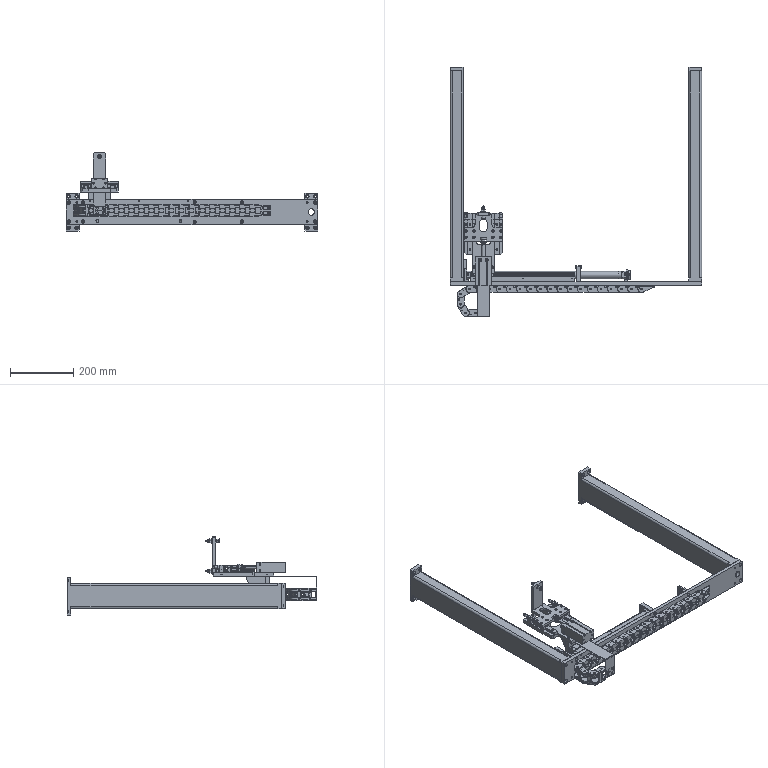Assembly | SolidWorks | mm | 74 component files | 74 solids | 4360 faces | box 795 x 790.5 x 247 mm | volume 3471055 mm3 | plane 2175 | cylinder 1835 | cone 314 | torus 28 | spline 8 | commonest cylinder face diameters 5.5 x192 22 x138 23 x130 3.4 x126 0.4 x126 2.444 x84 9.434 x84 5 x68
Bill of materials:
A0116 | 1 |  | Thick rectangular plate with an L-shaped side profile (a stepped ledge at one end), two chamfered corners on one long edge, one large and one medium through bore, a small face hole, and holes drilled into the narrow edge.
A0117 | 1 |  | Thin sheet-like L-shaped angle with a single rounded bend, a long flange and a shorter flange, and two small holes near the free end of the long flange.
A0131 | 1 |  | Plain rectangular block or thick bar with three round through holes on its main face in a triangular arrangement, one hole a different diameter from the other two.
A039 | 1 |  | Thick rectangular plate with two chamfered corners, a large through bore and a smaller bore, three small through holes along one edge, and three drilled holes in one narrow edge.
A066 | 1 |  | Long, thin flat bar with many through holes of several sizes spread along its length, including one larger hole near one end and small-hole groups near the ends and middle.
A067 | 2 |  | Long rectangular-section beam with a flat rectangular end plate at each end; the end plate has a large central bore, four corner through holes and two smaller blind holes; there are additional holes on the side near one end.
A091 | 1 |  | Long rectangular bar with a lengthwise rectangular groove along one face and a row of through holes of two or more sizes on the broad face.
1..2659899830.0 | 2 |  | Turned, stepped cylindrical part with a hexagonal collar near mid-length, a long cylindrical body, a slot across one end, and a small-diameter pin projecting from the other end with stepped shoulders.
A0106 | 2 |  | Solid rectangular block with one large round through hole near one end, passing through a pair of opposite faces.
A0110 | 1 |  | Rectangular plate with stepped faces (a transverse groove or step across one face and a small lip along the bottom edge), a pattern of about ten through holes including two larger bores, and two holes drilled into the top edge.
A0111 | 1 |  | Thick flat plate with a trapezoidal outline (one long diagonal edge, looking like a gusset), with two drilled holes in the top edge and two in the adjacent straight vertical edge.
A068 | 1 |  | Fork-shaped (U-slotted) thick plate: two parallel arms with a deep central slot that has rounded inner corners, a narrower tongue section at the base, chamfered shoulder corners, raised pads and steps at the arm ends, shallow lengthwise grooves along the arms, and many through holes of different sizes.
A069 | 1 |  | Flat plate with a roughly T-shaped outline. It has a central obround through-slot, eight round through-holes in two groups of four, and a T-shaped notch on one edge.
A070 | 1 |  | Axisymmetric spool or bushing shape: two flanges of different diameters joined by a smaller central hub, with a through-bore along the axis.
A071 | 1 |  | Thin rectangular plate with chamfered corners. It has two larger holes near the ends and two smaller holes near one end, beside notches in the long edges.
1.0.009603 | 1 |  | Rectangular block with two parallel narrow grooves running along its length. It has several holes on its faces and keyhole-like notches at the edges.
3..0..0.2 | 1 |  | Headed pin: a flat round disk head on a long cylindrical shank, which steps down to a smaller-diameter end section.
4..050.63 | 1 |  | Hexagonal prism with a large central round bore and chamfered (curved-edge) corners. Its shape matches a hex nut.
MANIFOLD_SOLID_BREP_100 | 2 |  | Rectangular block with an open channel through its underside, giving an inverted-U end profile. It has four holes on top and a seam line across the top near one end.
MANIFOLD_SOLID_BREP_99_1 | 2 |  | Straight bar of constant cross-section with three equally spaced holes through the top, rounded grooves along both sides, and chamfered corners.
1_2 | 2 |  | Elongated stepped turned part. It has a small flange at one end, cylindrical body sections, a knurled ring, and a hex section near the other end, with an axial bore at the flanged end.
2_2 | 2 |  | Axisymmetric stepped part: a cylindrical body with a rounded end and a small axial hole, a larger-diameter collar, a conical taper, a neck groove, and a small conical tip.
4_1 | 2 |  | Thin hexagonal ring with a large round bore and chamfered corners. Its shape matches a thin hex nut or lock-ring.
HGR15_1 | 1 |  | Long straight bar of constant cross-section with a shaped profile and a row of evenly spaced small holes along one side.
HGH15_2 | 1 |  | Rectangular prismatic block with a full-length open channel along one side, giving a C-shaped end profile. The top has a raised central section between lower stepped end sections. Generic shape resembles a linear-guide carriage block, but this is not confirmed.
10 | 1 |  | Link-like body made of two parallel stadium-shaped (obround) side plates joined by a central rectangular web, leaving an open rectangular window between the plates. At one end the plates are stepped outward (joggled). That end has a cylindrical boss or pin with a small bore; the other end has a plain through hole. Overall shape resembles a cable-carrier or chain link.
11 | 1 |  | Looks the same as the other link-like parts: two parallel stadium-shaped side plates joined by a central web with an open rectangular window, joggled plate ends, a cylindrical bored boss at one end and a through hole at the other.
12 | 1 |  | Looks the same as the other link-like parts: two parallel stadium-shaped side plates joined by a central web with an open rectangular window, joggled plate ends, a cylindrical bored boss at one end and a through hole at the other.
13 | 1 |  | Looks the same as the other link-like parts: two parallel stadium-shaped side plates joined by a central web with an open rectangular window, joggled plate ends, a cylindrical bored boss at one end and a through hole at the other.
14 | 1 |  | Looks the same as the other link-like parts: two parallel stadium-shaped side plates joined by a central web with an open rectangular window, joggled plate ends, a cylindrical bored boss at one end and a through hole at the other.
15 | 1 |  | Looks the same as the other link-like parts: two parallel stadium-shaped side plates joined by a central web with an open rectangular window, joggled plate ends, a cylindrical bored boss at one end and a through hole at the other.
16 | 1 |  | Looks the same as the other link-like parts: two parallel stadium-shaped side plates joined by a central web with an open rectangular window, joggled plate ends, a cylindrical bored boss at one end and a through hole at the other.
17 | 1 |  | Looks the same as the other link-like parts: two parallel stadium-shaped side plates joined by a central web with an open rectangular window, joggled plate ends, a cylindrical bored boss at one end and a through hole at the other.
18 | 1 |  | Looks the same as the other link-like parts: two parallel stadium-shaped side plates joined by a central web with an open rectangular window, joggled plate ends, a cylindrical bored boss at one end and a through hole at the other.
19 | 1 |  | Looks the same as the other link-like parts: two parallel stadium-shaped side plates joined by a central web with an open rectangular window, joggled plate ends, a cylindrical bored boss at one end and a through hole at the other.
20 | 1 |  | Looks the same as the other link-like parts: two parallel stadium-shaped side plates joined by a central web with an open rectangular window, joggled plate ends, a cylindrical bored boss at one end and a through hole at the other.
21 | 1 |  | Link-like frame: two parallel obround side plates joined by a central rectangular web, with a through-hole at one end and a short hollow cylindrical boss at the other.
22 | 1 |  | Link-like frame: two parallel obround side plates joined by a central rectangular web, with a through-hole at one end and a short hollow cylindrical boss at the other.
34 | 1 |  | Bent L-bracket: a tapered, teardrop-shaped flat flange with a round hole at its rounded end, and a perpendicular rectangular tab with two round holes rising from its straight edge.
35 | 1 |  | Bent L-bracket with a tapered teardrop flange and a perpendicular two-hole tab. Plan profile matches unnamed part, but the tab is bent the opposite way.
36 | 1 |  | Bent L-bracket: tapered teardrop flange with a central hole and several perimeter notches at the rounded end, plus a perpendicular two-hole tab along the flange's straight edge.
37 | 1 |  | Bent L-bracket with a notched teardrop flange and a perpendicular two-hole tab. Plan profile matches unnamed part, but the tab is bent the opposite way.
6 | 5 |  | Link-like frame: two parallel obround side plates joined by a central rectangular web, with a through-hole at one end and a short hollow cylindrical boss at the other.
7 | 1 |  | Link-like frame: two parallel obround side plates joined by a central rectangular web, with a through-hole at one end and a short hollow cylindrical boss at the other.
8 | 1 |  | Link-like frame: two parallel obround side plates joined by a central rectangular web, with a through-hole at one end and a short hollow cylindrical boss at the other.
9 | 1 |  | Link-like frame: two parallel obround side plates joined by a central rectangular web, with a through-hole at one end and a short hollow cylindrical boss at the other.
Mirror_A0116 | 1 |  | Thick rectangular plate with two chamfered corners on one long edge and three round through-holes of different sizes in the face. A stepped, L-shaped side profile forms a thicker lip along one end.
RMS20X400_0_Barrel | 1 |  | Straight thin-walled round tube with plain square-cut ends.
RMS20X50_Body | 1 |  | Rectangular prismatic block with a square end face containing a large circular bore along the long axis; concentric stepped rings or grooves surround the bore opening, and two small holes or features sit on the end face near the bore.
RMS20X50_FCV | 2 |  | Axially symmetric fitting-like body with a central hexagonal section and a cylindrical spigot on each side, chamfered at the outer ends, plus a central bore.
RMS20X50_Nut | 2 |  | Thin hexagonal nut-like ring with a large plain circular through-hole and chamfered corners on both faces.
RMS20X50_Piston | 1 |  | Solid stepped cylindrical shaft or pin: a large central cylinder with a smaller-diameter journal or stub at each end, a small shoulder step between them, and rounded or chamfered ends.
1 | 4 |  | Bolt-like part with a hexagonal head, a short cylindrical boss on the outer side of the head, a plain cylindrical shank with a chamfered tip, and a hexagonal socket recess in the shank end.
2 | 4 |  | Hexagonal nut-like body, thicker than part-02d4..., with a plain circular through-hole and chamfers on both faces.
Mates:
1. coincident | A066-2 face at (318.881, 0, 60) dir (0, 1, 0) | A067-6 face at (696.381, 0, 60) dir (0, -1, 0)
2. coincident | A066-2 face at (716.381, -12, 100) dir (1, 0, 0) | A067-6 face at (716.381, 12, 26) dir (1, 0, 0)
3. coincident | A066-2 face at (716.381, -12, 20) dir (0, 0, -1) | A067-6 face at (682.381, 12, 20) dir (0, 0, -1)
4. coincident | A066-2 face at (318.881, 0, 60) dir (0, 1, 0) | A067-7 face at (-58.619, 0, 60) dir (0, -1, 0)
5. coincident | A066-2 face at (716.381, -12, 100) dir (0, 0, 1) | A067-7 face at (-72.619, 12, 100) dir (0, 0, 1)
6. coincident | A066-2 face at (-78.619, -12, 100) dir (-1, 0, 0) | A067-7 face at (-78.619, 12, 26) dir (-1, 0, 0)
7. coincident | HandlingMechanism-2/A0110-1 face at (25.881, 41, 71.5) dir (0, -1, 0) | RMS_20X400_03-1/RMS20X50_Body-1 face at (60.881, 41, 22) dir (0, 1, 0)
8. coincident | HandlingMechanism-2/A0110-1 face at (60.881, 51.5, 20) dir (1, 0, 0) | RMS_20X400_03-1/RMS20X50_Body-1 face at (60.881, 40.5, 61) dir (1, 0, 0)
9. concentric | RMS_20X400_03-1/RMS20X400_0_Barrel-1 face at (463.381, 21, 41.5) dir (-1, 0, 0) r 11.5 | A0116-1 face at (-32.619, 21, 41.5) dir (1, 0, 0) r 10
10. coincident | A066-2 face at (318.881, 0, 60) dir (0, 1, 0) | A0116-1 face at (-20.619, 0, 100) dir (0, -1, 0)
11. coincident | RMS_20X400_03-1/RMS20X50_FCV-1 face at (-27.619, 21, 31.5) dir (-1, 0, 0) | A0116-1 face at (-27.619, 38.5, 100) dir (1, 0, 0)
12. concentric | RMS_20X400_03-1/RMS20X400_0_Barrel-1 face at (463.381, 21, 41.5) dir (-1, 0, 0) r 11.5 | Mirror_A0116-3 face at (483.381, 21, 41.5) dir (-1, 0, 0) r 10
13. coincident | A0116-1 face at (-32.619, 0, 20) dir (0, 0, -1) | Mirror_A0116-3 face at (483.381, 0, 20) dir (0, 0, -1)
14. coincident | RMS_20X400_03-1/RMS20X50_FCV-2 face at (478.381, 21, 51.5) dir (1, 0, 0) | Mirror_A0116-3 face at (478.381, 38.5, 100) dir (-1, 0, 0)
15. distance | HandlingMechanism-2/A071-1 plane at (25.881, 208.5, 187) dir (-1, 0, 0) | A067-7 face at (-38.619, 12, 26) dir (1, 0, 0)
16. distance | HandlingMechanism-2/A0110-1 face at (60.881, 51.5, 20) dir (0, 0, -1) | RMS_20X400_03-1/RMS20X50_Body-1 face at (60.881, 1.5, 21.5) dir (0, 0, -1)
17. distance | A066-2 face at (716.381, -12, 20) dir (0, 0, -1) | RMS_20X400_03-1/RMS20X50_Body-1 face at (60.881, 1.5, 21.5) dir (0, 0, -1)
18. coincident | A066-2 face at (318.881, -12, 60) dir (0, -1, 0) | MHPUS204-38-33-A-1/35-1 face at (568.833, -12, 81.7) dir (0, 1, 0)
19. distance | MHPUS204-38-33-A-1 plane at (-41.387, -64.533, 65) dir (0, 0, 1) | HandlingMechanism-2/CDU25-40A-A93(0_0)-2/1.0.009603-1 face at (36.881, 78.5, 135) dir (0, 0, -1)
20. coincident | HandlingMechanism-2/A068-1 face at (25.881, 120.5, 123) dir (0, 0, -1) | A0117-1 face at (45.881, -111.5, 123) dir (0, 0, 1)
21. coincident | HandlingMechanism-2/A0110-1 face at (25.881, 39.5, 71.5) dir (0, -1, 0) | A0117-1 face at (45.881, 39.5, 123) dir (0, 1, 0)
22. width | A0117-1 face at (45.881, -110, 121) dir (1, 0, 0) | A0117-1 face at (5.881, -109.5, 121) dir (-1, 0, 0) | HandlingMechanism-2/A068-1 face at (60.881, 24.5, 115) dir (1, 0, 0) | HandlingMechanism-2/A068-1 face at (-9.119, 24.5, 115) dir (-1, 0, 0)
23. concentric | Mirror_A0116-3 face at (483.381, 23.5, 75) dir (1, 0, 0) r 2.5 | USTH5-15-1/1-1 face at (484.735, 23.5, 75) dir (1, 0, 0) r 2.5
24. coincident | Mirror_A0116-3 face at (483.381, 0, 100) dir (1, 0, 0) | USTH5-15-1/2-1 face at (483.381, 21.5, 75) dir (-1, 0, 0)
25. concentric | A0116-1 face at (-32.619, 23.5, 75) dir (-1, 0, 0) r 2.5 | USTH5-15-2/1-1 face at (-33.974, 23.5, 75) dir (-1, 0, 0) r 2.5
26. coincident | A0116-1 face at (-32.619, 0, 100) dir (-1, 0, 0) | USTH5-15-2/2-1 face at (-32.619, 22.736, 76.848) dir (1, 0, 0)
27. coincident | A066-2 face at (318.881, 0, 60) dir (0, 1, 0) | A039-1 face at (333.381, 0, 100) dir (0, -1, 0)
28. distance | A039-1 face at (333.381, 25.5, 60) dir (1, 0, 0) | Mirror_A0116-3 face at (478.381, 38.5, 100) dir (-1, 0, 0)
29. coincident | A066-2 face at (716.381, -12, 100) dir (0, 0, 1) | A039-1 face at (333.381, 51, 100) dir (0, 0, 1)
30. coincident | USTH5-15-3/1-1 face at (316.381, 47.5, 90) dir (-1, 0, 0) | USTH5-15-4/1-1 face at (316.381, 47.5, 30) dir (-1, 0, 0)
31. concentric | A039-1 face at (333.381, 46, 30) dir (1, 0, 0) r 2.5 | USTH5-15-4/1-1 face at (328.635, 46, 30) dir (1, 0, 0) r 2.5
32. concentric | A039-1 face at (333.381, 46, 90) dir (1, 0, 0) r 2.5 | USTH5-15-3/1-1 face at (328.635, 46, 90) dir (1, 0, 0) r 2.5
33. coincident | A039-1 face at (321.381, 25.5, 60) dir (-1, 0, 0) | USTH5-15-3/1-1 face at (321.381, 49.65, 90) dir (1, 0, 0)
34. coincident | HandlingMechanism-2/A0110-1 face at (25.881, 41, 71.5) dir (0, -1, 0) | HGH15CA-1/HGH15_2-1 face at (6.181, 41, 92) dir (0, 1, 0)
35. coincident | HandlingMechanism-2/A0110-1 face at (60.881, 41, 66) dir (0, 0, 1) | HGH15CA-1/HGH15_2-1 face at (6.181, 35, 66) dir (0, 0, -1)
36. width | HGH15CA-1/HGH_15_ASM_3_ASM-1/HGR15_1-1 face at (315.381, 21.635, 76.177) dir (1, 0, 0) | HGH15CA-1/HGH_15_ASM_3_ASM-1/HGR15_1-1 face at (-14.619, 28, 83) dir (-1, 0, 0) | A0116-1 face at (-20.619, 8, 100) dir (1, 0, 0) | A039-1 face at (321.381, 25.5, 60) dir (-1, 0, 0)
37. width | HGH15CA-1/HGH15_2-1 face at (56.581, 28, 83) dir (1, 0, 0) | HGH15CA-1/HGH15_2-1 face at (-4.819, 28, 83) dir (-1, 0, 0) | HandlingMechanism-2/A0110-1 face at (-9.119, 51.5, 20) dir (-1, 0, 0) | HandlingMechanism-2/A0110-1 face at (60.881, 51.5, 20) dir (1, 0, 0)
38. coincident | A066-2 face at (318.881, 0, 60) dir (0, 1, 0) | A091-2 face at (150.381, 0, 83) dir (0, -1, 0)
39. coincident | HGH15CA-1/HGH_15_ASM_3_ASM-1/HGR15_1-1 face at (-14.619, 13.7, 75.5) dir (0, 0, -1) | A091-2 face at (-14.619, 13, 75.5) dir (0, 0, 1)
40. coincident | HGH15CA-1/HGH_15_ASM_3_ASM-1/HGR15_1-1 face at (315.381, 21.635, 76.177) dir (1, 0, 0) | A091-2 face at (315.381, 15, 100) dir (1, 0, 0)
41. coincident | A067-7 face at (-38.619, 12, 26) dir (1, 0, 0) | A0131-1 face at (-38.619, 56, 60) dir (-1, 0, 0)
42. coincident | A067-7 face at (-72.619, 12, 20) dir (0, 0, -1) | A0131-1 face at (-28.619, 41, 20) dir (0, 0, -1)
43. coincident | HandlingMechanism-2/A0110-1 face at (25.881, 41, 71.5) dir (0, -1, 0) | A0131-1 face at (-28.619, 41, 20) dir (0, -1, 0)
44. coincident | A039-1 face at (333.381, 25.5, 60) dir (1, 0, 0) | USTH5-15-3/2-1 face at (333.381, 44, 90) dir (-1, 0, 0)
45. concentric | A039-1 face at (333.381, 46, 90) dir (1, 0, 0) r 2.5 | USTH5-15-3/2-1 face at (336.581, 46, 90) dir (-1, 0, 0) r 2.5
46. coincident | A039-1 face at (333.381, 25.5, 60) dir (1, 0, 0) | USTH5-15-4/2-1 face at (333.381, 44, 30) dir (-1, 0, 0)
47. concentric | A039-1 face at (333.381, 46, 30) dir (1, 0, 0) r 2.5 | USTH5-15-4/2-1 face at (336.581, 46, 30) dir (-1, 0, 0) r 2.5
48. parallel | A069-1 face at (-48.143, -85.976, 28) dir (0, -1, 0) | A071-1 face at (11.857, -82.976, 58) dir (0, 1, 0)
49. width | A071-1 face at (-8.143, -92.976, 118) dir (-1, 0, 0) | A071-1 face at (31.857, -92.976, 118) dir (1, 0, 0) | A068-1 face at (-10.643, -90.976, -6) dir (1, 0, 0) | A068-1 face at (34.357, -90.976, -6) dir (-1, 0, 0)
50. coincident | A071-1 face at (11.857, -92.976, 58) dir (0, -1, 0) | MVPTN2-1/4_1-1 face at (9.652, -92.976, 12.718) dir (0, 1, 0)
51. concentric | A071-1 face at (11.857, -92.976, 10) dir (0, -1, 0) r 6 | MVPTN2-1/1_2-1 face at (11.857, -89.976, 10) dir (0, -1, 0) r 6
52. concentric | A071-1 face at (11.857, -92.976, 106) dir (0, -1, 0) r 6 | MVPTN2-3/1_2-1 face at (11.857, -89.976, 106) dir (0, -1, 0) r 6
53. coincident | A068-1 face at (11.857, 5.024, 4) dir (0, 0, 1) | A0106-1 face at (-43.143, -64.976, 4) dir (0, 0, -1)
54. coincident | A068-1 face at (-48.143, 101.024, 6) dir (-1, 0, 0) | A0106-1 face at (-48.143, -58.976, 4) dir (-1, 0, 0)
55. coincident | A068-1 face at (11.857, 5.024, 4) dir (0, 0, 1) | A0106-2 face at (66.857, -64.976, 4) dir (0, 0, -1)
56. coincident | A068-1 face at (71.857, 101.024, 6) dir (1, 0, 0) | A0106-2 face at (71.857, -58.976, 4) dir (1, 0, 0)
57. coincident | A068-1 face at (-48.143, -58.976, 4) dir (0, -1, 0) | A0106-2 face at (61.857, -58.976, 4) dir (0, 1, 0)
58. coincident | A068-1 face at (-48.143, -58.976, 4) dir (0, -1, 0) | A0106-1 face at (-48.143, -58.976, 4) dir (0, 1, 0)
59. coincident | A069-1 face at (1.857, -13.976, 13) dir (0, 1, 0) | A070-1 face at (11.857, -13.976, 22) dir (0, -1, 0)
60. concentric | A0106-2 face at (66.857, -58.976, 23) dir (0, 1, 0) r 4 | 1..2659899830.0-1 face at (66.857, -70.076, 23) dir (0, -1, 0) r 4
61. coincident | A0106-2 face at (61.857, -70.976, 4) dir (0, -1, 0) | 1..2659899830.0-1 face at (66.857, -70.976, 23) dir (0, 1, 0)
62. concentric | A0106-1 face at (-43.143, -58.976, 23) dir (0, 1, 0) r 4 | RB0805(0)-1/1..2659899830.0-1 face at (-43.143, -70.076, 23) dir (0, -1, 0) r 4
63. coincident | A0106-1 face at (-48.143, -70.976, 4) dir (0, -1, 0) | RB0805(0)-1/1..2659899830.0-1 face at (-43.143, -70.976, 23) dir (0, 1, 0)
64. distance | A071-1 face at (31.857, -92.976, 118) dir (0, 0, 1) | A069-1 face at (11.857, -44.476, 28) dir (0, 0, 1)
65. coincident | A068-1 face at (11.857, 5.024, -6) dir (0, 0, -1) | A0110-1 face at (-23.143, 74.024, -6) dir (0, 0, 1)
66. width | A069-1 face at (-48.143, -2.976, 28) dir (-1, 0, 0) | A069-1 face at (71.857, -2.976, 28) dir (1, 0, 0) | A068-1 face at (71.857, 101.024, 6) dir (1, 0, 0) | A068-1 face at (-48.143, 101.024, 6) dir (-1, 0, 0)
67. concentric | A070-1 face at (11.857, 1.024, 22) dir (0, -1, 0) r 9.75 | CDU25-40A-A93(0_0)-2/3..0..0.2-1 face at (11.857, -2.592, 22) dir (0, 1, 0) r 4
68. coincident | A070-1 face at (11.857, 1.024, 22) dir (0, 1, 0) | CDU25-40A-A93(0_0)-2/4..050.63-1 face at (10.204, 1.024, 17.017) dir (0, -1, 0)
69. coincident | MGN15C-5/MANIFOLD_SOLID_BREP_100-2 face at (-46.643, -37.826, 19.75) dir (0, 0, 1) | MGN15C-6/MANIFOLD_SOLID_BREP_100-2 face at (38.357, -37.826, 19.75) dir (0, 0, 1)
70. coincident | A068-1 face at (11.857, 5.024, 4) dir (0, 0, 1) | MGN15C-5/MANIFOLD_SOLID_BREP_99_1-1 face at (-38.143, -70.976, 4) dir (0, 0, -1)
71. coincident | A068-1 face at (-38.143, 39.024, 4) dir (1, 0, 0) | MGN15C-5/MANIFOLD_SOLID_BREP_99_1-1 face at (-38.143, -70.976, 9) dir (-1, 0, 0)
72. coincident | A068-1 face at (61.857, 39.024, 4) dir (-1, 0, 0) | MGN15C-6/MANIFOLD_SOLID_BREP_99_1-1 face at (61.857, -70.976, 4) dir (1, 0, 0)
73. coincident | A069-1 face at (11.857, -44.476, 20) dir (0, 0, -1) | MGN15C-5/MANIFOLD_SOLID_BREP_100-2 face at (-46.643, -45.526, 20) dir (0, 0, 1)
74. coincident | MGN15C-5/MANIFOLD_SOLID_BREP_100-2 face at (-14.643, -3.426, 12) dir (0, 1, 0) | MGN15C-6/MANIFOLD_SOLID_BREP_100-2 face at (70.357, -3.426, 12) dir (0, 1, 0)
75. coincident | A071-1 face at (11.857, -92.976, 58) dir (0, -1, 0) | MVPTN2-3/4_1-1 face at (11.669, -92.976, 102.505) dir (0, 1, 0)
76. width | A0110-1 face at (-23.143, 74.024, -109) dir (-1, 0, 0) | A0110-1 face at (46.857, 74.024, -109) dir (1, 0, 0) | A068-1 face at (46.857, 101.024, -14) dir (1, 0, 0) | A068-1 face at (-23.143, 101.024, -14) dir (-1, 0, 0)
77. width | A0111-2 face at (5.857, 44.024, -48.5) dir (-1, 0, 0) | A0111-2 face at (17.857, 44.024, -48.5) dir (1, 0, 0) | A0110-1 face at (-23.143, 74.024, -109) dir (-1, 0, 0) | A0110-1 face at (46.857, 74.024, -109) dir (1, 0, 0)
78. distance | CDU25-40A-A93(0_0)-2/1.0.009603-1 face at (11.857, 47.024, 22) dir (0, -1, 0) | A068-1 face at (-48.143, -90.976, 6) dir (0, -1, 0)
79. coincident | A068-1 face at (11.857, 5.024, 6) dir (0, 0, 1) | CDU25-40A-A93(0_0)-2/1.0.009603-1 face at (25.857, 47.024, 6) dir (0, 0, -1)
80. width | CDU25-40A-A93(0_0)-2/1.0.009603-1 face at (-13.143, 47.024, 38) dir (-1, 0, 0) | CDU25-40A-A93(0_0)-2/1.0.009603-1 face at (36.857, 47.024, 6) dir (1, 0, 0) | A068-1 face at (71.857, 101.024, 6) dir (1, 0, 0) | A068-1 face at (-48.143, 101.024, 6) dir (-1, 0, 0)
81. coincident | A069-1 face at (30.857, -82.976, 38) dir (0, -1, 0) | A071-1 face at (11.857, -82.976, 58) dir (0, 1, 0)
82. coincident | A0110-1 face at (11.857, 74.024, -57.5) dir (0, -1, 0) | A0111-2 face at (17.857, 74.024, -91) dir (0, 1, 0)
83. coincident | A068-1 face at (11.857, 5.024, -6) dir (0, 0, -1) | A0111-2 face at (17.857, 14.024, -6) dir (0, 0, 1)
84. width | A0111-2 face at (17.857, 44.024, -48.5) dir (1, 0, 0) | A0111-2 face at (5.857, 44.024, -48.5) dir (-1, 0, 0) | A0110-1 face at (-23.143, 74.024, -109) dir (-1, 0, 0) | A0110-1 face at (46.857, 74.024, -109) dir (1, 0, 0)
85. distance | A0110-1 face at (11.857, 86.024, -57.5) dir (0, 1, 0) | A068-1 face at (71.857, 39.024, -14) dir (0, 1, 0)
86. concentric | A069-1 face at (66.857, -34.476, 28) dir (0, 0, 1) r 2.15 | MGN15C-6/MANIFOLD_SOLID_BREP_100-2 face at (66.857, -34.476, 20) dir (0, 0, -1) r 1.5
87. concentric | A069-1 face at (66.857, -14.476, 28) dir (0, 0, 1) r 2.15 | MGN15C-6/MANIFOLD_SOLID_BREP_100-2 face at (66.857, -14.476, 20) dir (0, 0, -1) r 1.5
88. concentric | A069-1 face at (-43.143, -34.476, 28) dir (0, 0, 1) r 2.15 | MGN15C-5/MANIFOLD_SOLID_BREP_100-2 face at (-43.143, -34.476, 20) dir (0, 0, -1) r 1.5
89. concentric | A069-1 face at (-43.143, -14.476, 28) dir (0, 0, 1) r 2.15 | MGN15C-5/MANIFOLD_SOLID_BREP_100-2 face at (-43.143, -14.476, 20) dir (0, 0, -1) r 1.5
90. coincident | A068-1 face at (-48.143, 39.024, -14) dir (0, 1, 0) | MGN15C-5/MANIFOLD_SOLID_BREP_99_1-1 face at (-29.643, 39.024, 4) dir (0, 1, 0)
91. coincident | A068-1 face at (71.857, 39.024, -14) dir (0, 1, 0) | MGN15C-6/MANIFOLD_SOLID_BREP_99_1-1 face at (55.357, 39.024, 4) dir (0, 1, 0)
92. concentric | 3..0..0.2-1 face at (-38.432, 42.862, 93.705) dir (0, 0, -1) r 4 | 4..050.63-1 face at (-38.432, 42.862, 87.588) dir (0, 0, -1) r 3.324
93. coincident | 3..0..0.2-1 edge at (-38.432, 42.862, 85.088) dir (0, 0, -1) r 4 | 4..050.63-1 face at (-38.432, 48.112, 85.088) dir (0, 0, -1)
94. concentric | 1.0.009603-1 face at (-38.432, 42.862, 27.213) dir (0, 0, -1) r 5 | 3..0..0.2-1 face at (-38.432, 42.862, 49.213) dir (0, 0, -1) r 5
95. distance | 3..0..0.2-1 face at (-30.196, 45.819, 14.338) dir (0, 0, 1) | 1.0.009603-1 face at (-38.432, 49.112, -30.662) dir (0, 0, 1)
96. coincident | MANIFOLD_SOLID_BREP_99_1-1 face at (21.631, 13, 143.222) dir (0, 1, 0) | MANIFOLD_SOLID_BREP_100-2 face at (21.631, 13, 160.355) dir (0, -1, 0)
97. width | MANIFOLD_SOLID_BREP_100-2 face at (-1.869, 7, 126.405) dir (-1, 0, 0) | MANIFOLD_SOLID_BREP_100-2 face at (30.131, 19, 126.405) dir (1, 0, 0) | MANIFOLD_SOLID_BREP_99_1-1 face at (21.631, 3, 143.222) dir (1, 0, 0) | MANIFOLD_SOLID_BREP_99_1-1 face at (6.631, 8, 143.222) dir (-1, 0, 0)
98. concentric | 1_2-1 face at (8.638, 25.061, 13.204) dir (0, -1, 0) r 6 | 4_1-1 face at (8.638, 20.061, 13.204) dir (0, 1, 0) r 5.458
99. coincident | 1_2-1 face at (11.638, 18.061, 13.204) dir (0, 1, 0) | 4_1-1 face at (12.138, 18.061, 13.204) dir (0, -1, 0)
100. concentric | 1_2-1 face at (8.638, 6.561, 13.204) dir (0, -1, 0) r 2 | 2_2-1 face at (8.638, 6.411, 13.204) dir (0, -1, 0) r 1.6
101. coincident | 1_2-1 face at (10.638, 4.561, 13.204) dir (0, -1, 0) | 2_2-1 face at (10.438, 4.561, 13.204) dir (0, 1, 0)
102. width | HGH15_2-1 face at (13.858, 7, 25.799) dir (1, 0, 0) | HGH15_2-1 face at (-20.142, 12, 25.799) dir (-1, 0, 0) | HGH_15_ASM_3_ASM-1/HGR15_1-1 face at (-10.642, -11.757, -79.451) dir (-1, 0, 0) | HGH_15_ASM_3_ASM-1/HGR15_1-1 face at (4.358, -14.3, -79.451) dir (1, 0, 0)
103. coincident | HGH_15_ASM_3_ASM-1/HGR15_1-1 face at (1.907, 0, -79.451) dir (0, 1, 0) | HGH15_2-1 face at (-8.191, 0, 25.799) dir (0, -1, 0)
104. coincident | 34-1 face at (567.22, 52.533, -16.7) dir (0, 1, 0) | 35-1 face at (610.22, 52.533, 16.7) dir (0, 1, 0)
105. concentric | 22-1 face at (567.22, 41.533, -14.7) dir (0, 0, 1) r 2.75 | 34-1 face at (567.22, 41.533, -16.7) dir (0, 0, -1) r 2.75
106. concentric | 22-1 face at (567.22, 41.533, 14.7) dir (0, 0, -1) r 2.75 | 35-1 face at (567.22, 41.533, 16.7) dir (0, 0, 1) r 2.75
107. concentric | 6-2 face at (-5.032, -6.773, 14.4) dir (0, 0, -1) r 2.75 | 6-3 face at (-5.032, -6.773, -20) dir (0, 0, -1) r 2.75
108. concentric | 6-2 face at (11, -34.467, -20.3) dir (0, 0, -1) r 2.75 | 6-4 face at (11, -34.467, 14.7) dir (0, 0, -1) r 2.75
109. concentric | 36-1 face at (43, -34.467, -15) dir (0, 0, -1) r 2.75 | 6-4 face at (43, -34.467, -20) dir (0, 0, -1) r 2.75
110. coincident | 6-2 face at (16.511, -43.987, 14.7) dir (0, 0, -1) | 6-4 face at (54, -34.467, 14.7) dir (0, 0, 1)
111. concentric | 6-1 face at (23.22, 41.533, -20) dir (0, 0, -1) r 2.75 | 6-5 face at (23.22, 41.533, -14.7) dir (0, 0, 1) r 2.75
112. coincident | 6-1 face at (12.22, 52.533, -20) dir (0, 0, -1) | 6-5 face at (-19.381, 29.074, -20) dir (0, 0, -1)
113. concentric | 6-3 face at (-4.31, 25.219, -14.7) dir (0, 0, 1) r 2.75 | 6-5 face at (-4.31, 25.219, -20) dir (0, 0, -1) r 2.75
114. coincident | 37-1 face at (43, -45.467, 15) dir (0, 0, 1) | 6-4 face at (54, -34.467, 15) dir (0, 0, -1)
115. coincident | 36-1 face at (86, -45.467, -15) dir (0, -1, 0) | 6-4 face at (29.909, -45.467, 14.6) dir (0, -1, 0)
116. distance | RMS20X50_FCV-1 plane at (0, 0, 0) dir (1, 0, 0) | RMS_20X400_0_dummy-1 plane at (0, 0, 0) dir (-1, 0, 0)
117. coincident | RMS_20X400_0_dummy-1 axis at (-80.9, 0, 0) dir (1, 0, 0) | RMS20X50_FCV-1 axis at (80.9, 0, 0) dir (-1, 0, 0)
118. coincident | RMS_20X400_0_dummy-1 axis at (-80.9, 0, 0) dir (1, 0, 0) | RMS20X50_FCV-1 axis at (80.9, 0, 0) dir (-1, 0, 0)
119. coincident | RMS_20X400_0_dummy-1 axis at (-80.9, 0, 0) dir (1, 0, 0) | RMS20X50_FCV-1 axis at (80.9, 0, 0) dir (-1, 0, 0)
120. angle | RMS20X50_FCV-1 plane at (0, 0, 0) dir (0, 0, -1) | RMS_20X400_0_dummy-1 plane at (0, 0, 0) dir (0, 0, -1)
121. distance | RMS20X400_0_Barrel-1 plane at (0, 0, 0) dir (-1, 0, 0) | RMS20X50_FCV-1 plane at (0, 0, 0) dir (1, 0, 0)
122. coincident | RMS20X50_FCV-1 axis at (80.9, 0, 0) dir (-1, 0, 0) | RMS20X400_0_Barrel-1 axis at (-80.9, 0, 0) dir (1, 0, 0)
123. coincident | RMS20X50_FCV-1 axis at (80.9, 0, 0) dir (-1, 0, 0) | RMS20X400_0_Barrel-1 axis at (-80.9, 0, 0) dir (1, 0, 0)
124. coincident | RMS20X50_FCV-1 axis at (80.9, 0, 0) dir (-1, 0, 0) | RMS20X400_0_Barrel-1 axis at (-80.9, 0, 0) dir (1, 0, 0)
125. angle | RMS20X400_0_Barrel-1 plane at (0, 0, 0) dir (0, 0, -1) | RMS20X50_FCV-1 plane at (0, 0, 0) dir (0, 0, -1)
126. distance | RMS20X50_FCV-2 plane at (476, 0, 0) dir (-1, 0, 0) | RMS20X400_0_Barrel-1 plane at (476, 0, 0) dir (1, 0, 0)
127. coincident | RMS20X400_0_Barrel-1 axis at (80.9, 0, 0) dir (-1, 0, 0) | RMS20X50_FCV-2 axis at (395.1, 0, 0) dir (1, 0, 0)
128. coincident | RMS20X400_0_Barrel-1 axis at (80.9, 0, 0) dir (-1, 0, 0) | RMS20X50_FCV-2 axis at (395.1, 0, 0) dir (1, 0, 0)
129. coincident | RMS20X400_0_Barrel-1 axis at (80.9, 0, 0) dir (-1, 0, 0) | RMS20X50_FCV-2 axis at (395.1, 0, 0) dir (1, 0, 0)
130. angle | RMS20X50_FCV-2 plane at (476, 0, 0) dir (0, 0, -1) | RMS20X400_0_Barrel-1 plane at (0, 0, 0) dir (0, 0, -1)
131. distance | RMS20X50_Nut-1 plane at (504, 0, 0) dir (-1, 0, 0) | RMS20X50_FCV-2 plane at (491, 0, 0) dir (1, 0, 0)
132. coincident | RMS20X50_FCV-2 axis at (556.9, 0, 0) dir (-1, 0, 0) | RMS20X50_Nut-1 axis at (423.1, 0, 0) dir (1, 0, 0)
133. coincident | RMS20X50_FCV-2 axis at (556.9, 0, 0) dir (-1, 0, 0) | RMS20X50_Nut-1 axis at (423.1, 0, 0) dir (1, 0, 0)
134. coincident | RMS20X50_FCV-2 axis at (556.9, 0, 0) dir (-1, 0, 0) | RMS20X50_Nut-1 axis at (423.1, 0, 0) dir (1, 0, 0)
135. angle | RMS20X50_Nut-1 plane at (504, 0, 0) dir (0, 0, -1) | RMS20X50_FCV-2 plane at (476, 0, 0) dir (0, 0, -1)
136. distance | RMS20X50_Body-1 plane at (7.5, 0, 0) dir (-1, 0, 0) | RMS20X400_0_Barrel-1 plane at (5, 0, 0) dir (1, 0, 0)
137. coincident | RMS20X400_0_Barrel-1 axis at (80.9, 0, 0) dir (-1, 0, 0) | RMS20X50_Body-1 axis at (-73.4, 0, 0) dir (1, 0, 0)
138. coincident | RMS20X400_0_Barrel-1 axis at (80.9, 0, 0) dir (-1, 0, 0) | RMS20X50_Body-1 axis at (-73.4, 0, 0) dir (1, 0, 0)
139. coincident | RMS20X400_0_Barrel-1 axis at (80.9, 0, 0) dir (-1, 0, 0) | RMS20X50_Body-1 axis at (-73.4, 0, 0) dir (1, 0, 0)
140. angle | RMS20X50_Body-1 plane at (7.5, 0, 0) dir (0, 0, -1) | RMS20X400_0_Barrel-1 plane at (0, 0, 0) dir (0, 0, -1)
141. distance | RMS20X50_Piston-1 plane at (12.5, 0, 0) dir (-1, 0, 0) | RMS20X50_Body-1 plane at (12.5, 0, 0) dir (1, 0, 0)
142. coincident | RMS20X50_Body-1 axis at (88.4, 0, 0) dir (-1, 0, 0) | RMS20X50_Piston-1 axis at (-68.4, 0, 0) dir (1, 0, 0)
143. coincident | RMS20X50_Body-1 axis at (88.4, 0, 0) dir (-1, 0, 0) | RMS20X50_Piston-1 axis at (-68.4, 0, 0) dir (1, 0, 0)
144. coincident | RMS20X50_Body-1 axis at (88.4, 0, 0) dir (-1, 0, 0) | RMS20X50_Piston-1 axis at (-68.4, 0, 0) dir (1, 0, 0)
145. angle | RMS20X50_Piston-1 plane at (12.5, 0, 0) dir (0, 0, -1) | RMS20X50_Body-1 plane at (7.5, 0, 0) dir (0, 0, -1)
146. distance | RMS20X50_Nut-2 plane at (-28, 0, 0) dir (1, 0, 0) | RMS20X50_FCV-1 plane at (-15, 0, 0) dir (-1, 0, 0)
147. coincident | RMS20X50_FCV-1 axis at (-80.9, 0, 0) dir (1, 0, 0) | RMS20X50_Nut-2 axis at (52.9, 0, 0) dir (-1, 0, 0)
148. coincident | RMS20X50_FCV-1 axis at (-80.9, 0, 0) dir (1, 0, 0) | RMS20X50_Nut-2 axis at (52.9, 0, 0) dir (-1, 0, 0)
149. coincident | RMS20X50_FCV-1 axis at (-80.9, 0, 0) dir (1, 0, 0) | RMS20X50_Nut-2 axis at (52.9, 0, 0) dir (-1, 0, 0)
150. angle | RMS20X50_Nut-2 plane at (-28, 0, 0) dir (0, 0, -1) | RMS20X50_FCV-1 plane at (0, 0, 0) dir (0, 0, -1)